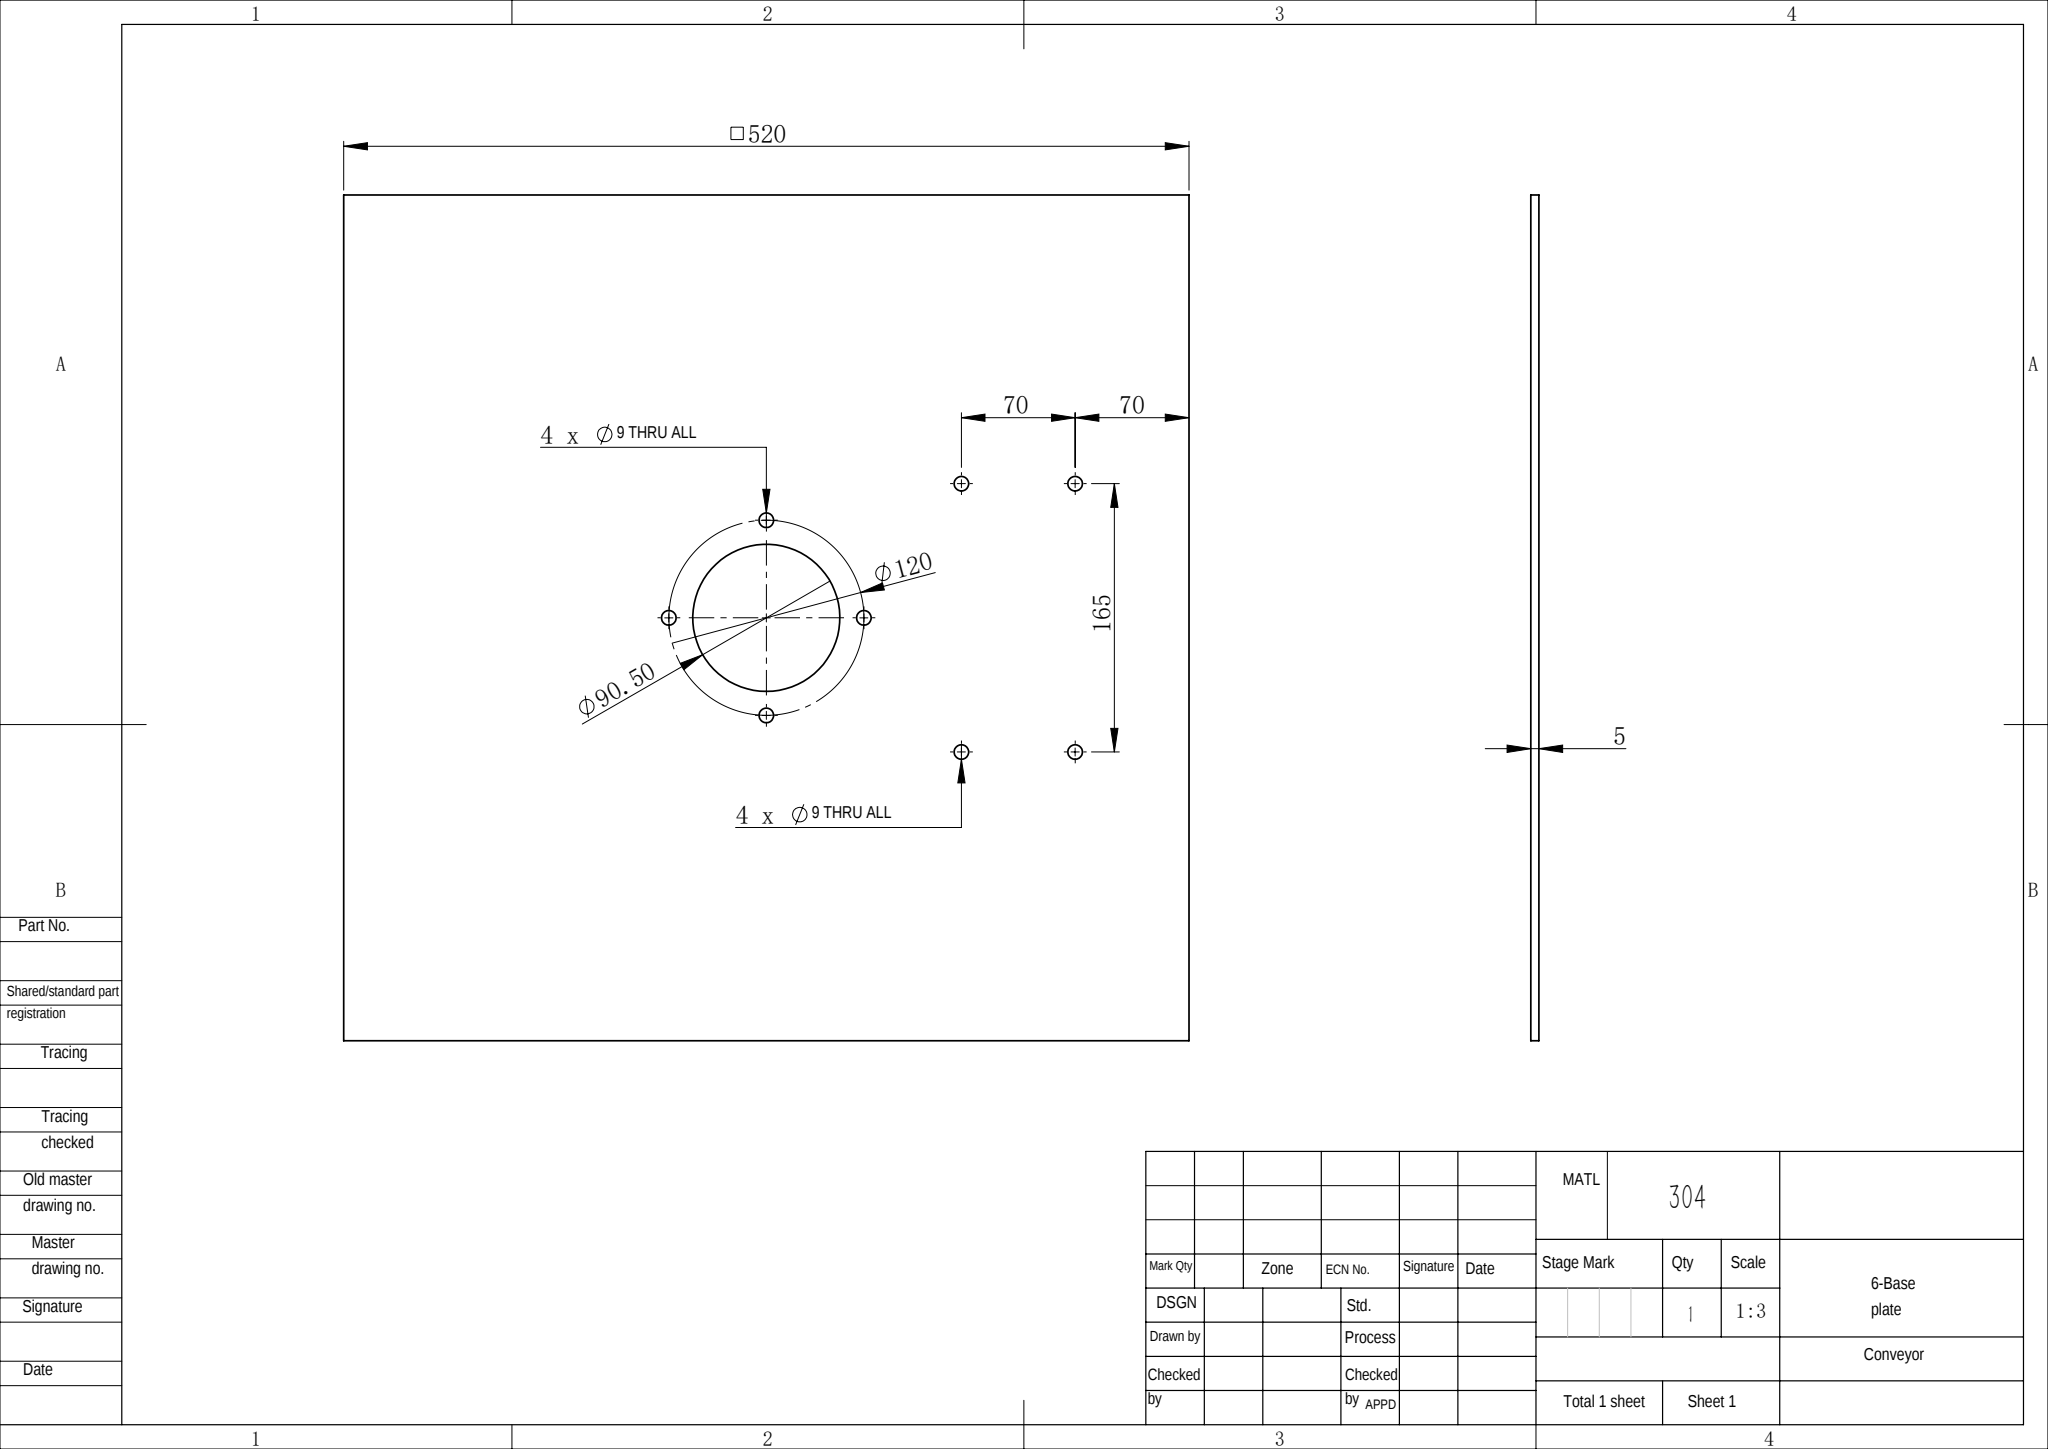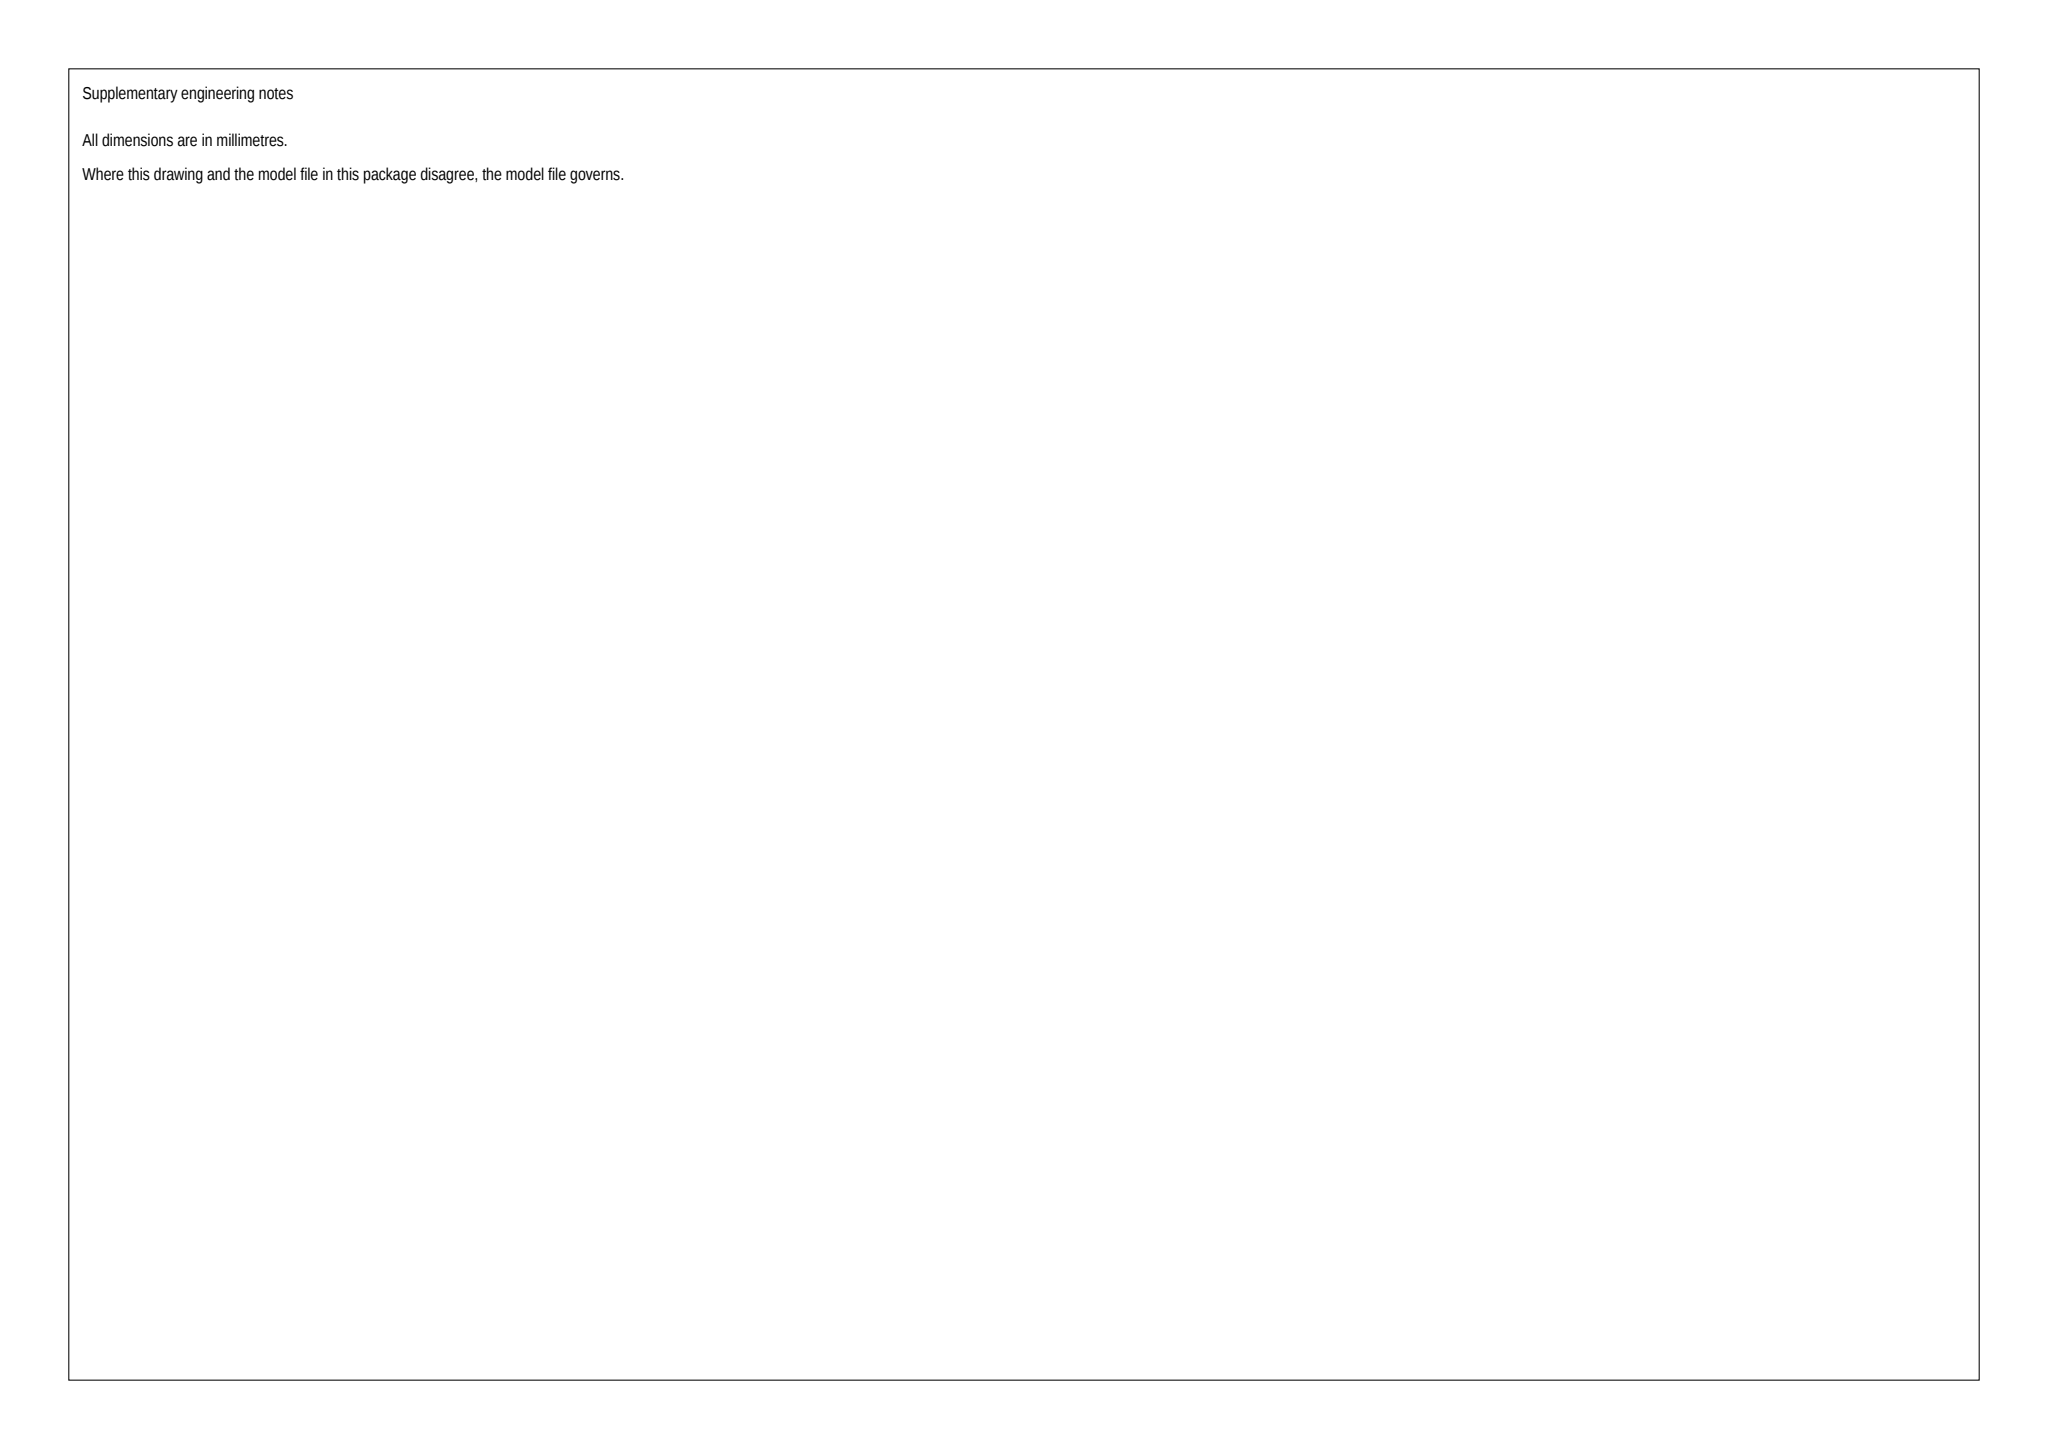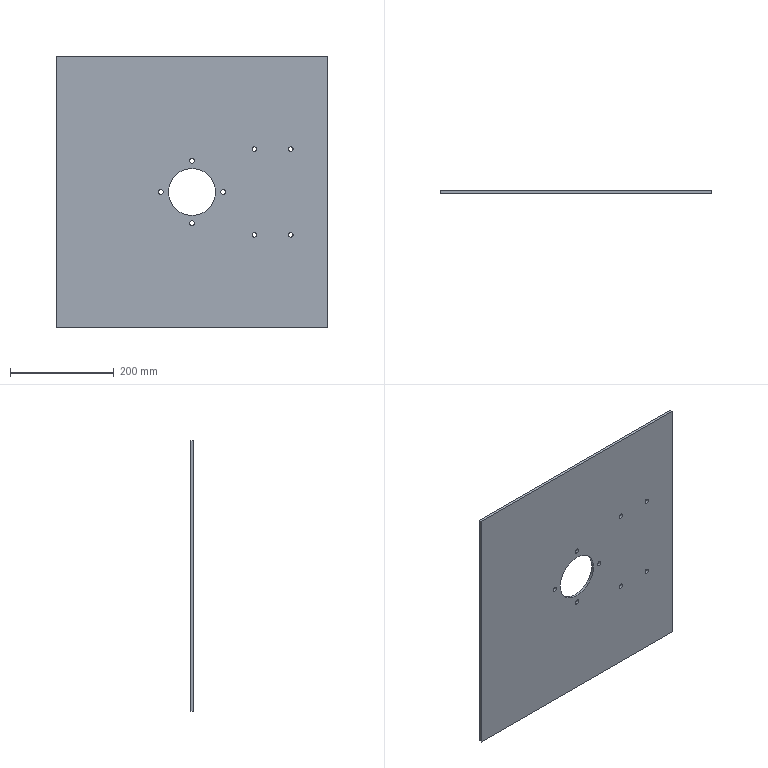Part | SolidWorks | mm | material 304 | 1 solid | 24 faces | box 520 x 5 x 520 mm | volume 1317292 mm3 | cylinder 18 | plane 6 | commonest cylinder face diameters 9 x16 90.5 x2
STEP:
#1=CARTESIAN_POINT('',(120.,-5.,-87.));
#2=VERTEX_POINT('',#1);
#3=CARTESIAN_POINT('',(120.,-5.,-78.));
#4=VERTEX_POINT('',#3);
#5=CARTESIAN_POINT('',(120.,-5.,-82.5));
#6=DIRECTION('',(0.,1.,0.));
#7=DIRECTION('',(0.,0.,1.));
#8=AXIS2_PLACEMENT_3D('',#5,#6,#7);
#9=CIRCLE('',#8,4.5);
#10=EDGE_CURVE('',#2,#4,#9,.T.);
#11=ORIENTED_EDGE('',*,*,#10,.F.);
#12=CARTESIAN_POINT('',(120.,-0.,-87.));
#13=VERTEX_POINT('',#12);
#14=CARTESIAN_POINT('',(120.,0.,-87.));
#15=DIRECTION('',(0.,1.,0.));
#16=VECTOR('',#15,1000.);
#17=LINE('',#14,#16);
#18=EDGE_CURVE('',#2,#13,#17,.T.);
#19=ORIENTED_EDGE('',*,*,#18,.T.);
#20=CARTESIAN_POINT('',(120.,-0.,-78.));
#21=VERTEX_POINT('',#20);
#22=CARTESIAN_POINT('',(120.,-0.,-82.5));
#23=DIRECTION('',(0.,1.,0.));
#24=DIRECTION('',(0.,0.,1.));
#25=AXIS2_PLACEMENT_3D('',#22,#23,#24);
#26=CIRCLE('',#25,4.5);
#27=EDGE_CURVE('',#13,#21,#26,.T.);
#28=ORIENTED_EDGE('',*,*,#27,.T.);
#29=CARTESIAN_POINT('',(120.,0.,-78.));
#30=DIRECTION('',(0.,1.,0.));
#31=VECTOR('',#30,1000.);
#32=LINE('',#29,#31);
#33=EDGE_CURVE('',#4,#21,#32,.T.);
#34=ORIENTED_EDGE('',*,*,#33,.F.);
#35=EDGE_LOOP('',(#11,#19,#28,#34));
#36=FACE_OUTER_BOUND('',#35,.T.);
#37=CARTESIAN_POINT('',(120.,0.,-82.5));
#38=DIRECTION('',(0.,1.,0.));
#39=DIRECTION('',(0.,0.,1.));
#40=AXIS2_PLACEMENT_3D('',#37,#38,#39);
#41=CYLINDRICAL_SURFACE('',#40,4.5);
#42=ADVANCED_FACE('',(#36),#41,.F.);
#43=CARTESIAN_POINT('',(190.,-5.,78.));
#44=VERTEX_POINT('',#43);
#45=CARTESIAN_POINT('',(190.,-5.,87.));
#46=VERTEX_POINT('',#45);
#47=CARTESIAN_POINT('',(190.,-5.,82.5));
#48=DIRECTION('',(0.,1.,0.));
#49=DIRECTION('',(0.,0.,1.));
#50=AXIS2_PLACEMENT_3D('',#47,#48,#49);
#51=CIRCLE('',#50,4.5);
#52=EDGE_CURVE('',#44,#46,#51,.T.);
#53=ORIENTED_EDGE('',*,*,#52,.F.);
#54=CARTESIAN_POINT('',(190.,-0.,78.));
#55=VERTEX_POINT('',#54);
#56=CARTESIAN_POINT('',(190.,0.,78.));
#57=DIRECTION('',(0.,1.,0.));
#58=VECTOR('',#57,1000.);
#59=LINE('',#56,#58);
#60=EDGE_CURVE('',#44,#55,#59,.T.);
#61=ORIENTED_EDGE('',*,*,#60,.T.);
#62=CARTESIAN_POINT('',(190.,-0.,87.));
#63=VERTEX_POINT('',#62);
#64=CARTESIAN_POINT('',(190.,-0.,82.5));
#65=DIRECTION('',(0.,1.,0.));
#66=DIRECTION('',(0.,0.,1.));
#67=AXIS2_PLACEMENT_3D('',#64,#65,#66);
#68=CIRCLE('',#67,4.5);
#69=EDGE_CURVE('',#55,#63,#68,.T.);
#70=ORIENTED_EDGE('',*,*,#69,.T.);
#71=CARTESIAN_POINT('',(190.,0.,87.));
#72=DIRECTION('',(0.,1.,0.));
#73=VECTOR('',#72,1000.);
#74=LINE('',#71,#73);
#75=EDGE_CURVE('',#46,#63,#74,.T.);
#76=ORIENTED_EDGE('',*,*,#75,.F.);
#77=EDGE_LOOP('',(#53,#61,#70,#76));
#78=FACE_OUTER_BOUND('',#77,.T.);
#79=CARTESIAN_POINT('',(190.,0.,82.5));
#80=DIRECTION('',(0.,1.,0.));
#81=DIRECTION('',(0.,0.,1.));
#82=AXIS2_PLACEMENT_3D('',#79,#80,#81);
#83=CYLINDRICAL_SURFACE('',#82,4.5);
#84=ADVANCED_FACE('',(#78),#83,.F.);
#85=CARTESIAN_POINT('',(190.,-5.,-87.));
#86=VERTEX_POINT('',#85);
#87=CARTESIAN_POINT('',(190.,-5.,-78.));
#88=VERTEX_POINT('',#87);
#89=CARTESIAN_POINT('',(190.,-5.,-82.5));
#90=DIRECTION('',(0.,1.,0.));
#91=DIRECTION('',(0.,0.,1.));
#92=AXIS2_PLACEMENT_3D('',#89,#90,#91);
#93=CIRCLE('',#92,4.5);
#94=EDGE_CURVE('',#86,#88,#93,.T.);
#95=ORIENTED_EDGE('',*,*,#94,.F.);
#96=CARTESIAN_POINT('',(190.,-0.,-87.));
#97=VERTEX_POINT('',#96);
#98=CARTESIAN_POINT('',(190.,0.,-87.));
#99=DIRECTION('',(0.,1.,0.));
#100=VECTOR('',#99,1000.);
#101=LINE('',#98,#100);
#102=EDGE_CURVE('',#86,#97,#101,.T.);
#103=ORIENTED_EDGE('',*,*,#102,.T.);
#104=CARTESIAN_POINT('',(190.,-0.,-78.));
#105=VERTEX_POINT('',#104);
#106=CARTESIAN_POINT('',(190.,-0.,-82.5));
#107=DIRECTION('',(0.,1.,0.));
#108=DIRECTION('',(0.,0.,1.));
#109=AXIS2_PLACEMENT_3D('',#106,#107,#108);
#110=CIRCLE('',#109,4.5);
#111=EDGE_CURVE('',#97,#105,#110,.T.);
#112=ORIENTED_EDGE('',*,*,#111,.T.);
#113=CARTESIAN_POINT('',(190.,0.,-78.));
#114=DIRECTION('',(0.,1.,0.));
#115=VECTOR('',#114,1000.);
#116=LINE('',#113,#115);
#117=EDGE_CURVE('',#88,#105,#116,.T.);
#118=ORIENTED_EDGE('',*,*,#117,.F.);
#119=EDGE_LOOP('',(#95,#103,#112,#118));
#120=FACE_OUTER_BOUND('',#119,.T.);
#121=CARTESIAN_POINT('',(190.,0.,-82.5));
#122=DIRECTION('',(0.,1.,0.));
#123=DIRECTION('',(0.,0.,1.));
#124=AXIS2_PLACEMENT_3D('',#121,#122,#123);
#125=CYLINDRICAL_SURFACE('',#124,4.5);
#126=ADVANCED_FACE('',(#120),#125,.F.);
#127=CARTESIAN_POINT('',(120.,-5.,78.));
#128=VERTEX_POINT('',#127);
#129=CARTESIAN_POINT('',(120.,-5.,87.));
#130=VERTEX_POINT('',#129);
#131=CARTESIAN_POINT('',(120.,-5.,82.5));
#132=DIRECTION('',(0.,1.,0.));
#133=DIRECTION('',(0.,0.,1.));
#134=AXIS2_PLACEMENT_3D('',#131,#132,#133);
#135=CIRCLE('',#134,4.5);
#136=EDGE_CURVE('',#128,#130,#135,.T.);
#137=ORIENTED_EDGE('',*,*,#136,.F.);
#138=CARTESIAN_POINT('',(120.,-0.,78.));
#139=VERTEX_POINT('',#138);
#140=CARTESIAN_POINT('',(120.,0.,78.));
#141=DIRECTION('',(0.,1.,0.));
#142=VECTOR('',#141,1000.);
#143=LINE('',#140,#142);
#144=EDGE_CURVE('',#128,#139,#143,.T.);
#145=ORIENTED_EDGE('',*,*,#144,.T.);
#146=CARTESIAN_POINT('',(120.,-0.,87.));
#147=VERTEX_POINT('',#146);
#148=CARTESIAN_POINT('',(120.,-0.,82.5));
#149=DIRECTION('',(0.,1.,0.));
#150=DIRECTION('',(0.,0.,1.));
#151=AXIS2_PLACEMENT_3D('',#148,#149,#150);
#152=CIRCLE('',#151,4.5);
#153=EDGE_CURVE('',#139,#147,#152,.T.);
#154=ORIENTED_EDGE('',*,*,#153,.T.);
#155=CARTESIAN_POINT('',(120.,0.,87.));
#156=DIRECTION('',(0.,1.,0.));
#157=VECTOR('',#156,1000.);
#158=LINE('',#155,#157);
#159=EDGE_CURVE('',#130,#147,#158,.T.);
#160=ORIENTED_EDGE('',*,*,#159,.F.);
#161=EDGE_LOOP('',(#137,#145,#154,#160));
#162=FACE_OUTER_BOUND('',#161,.T.);
#163=CARTESIAN_POINT('',(120.,0.,82.5));
#164=DIRECTION('',(0.,1.,0.));
#165=DIRECTION('',(0.,0.,1.));
#166=AXIS2_PLACEMENT_3D('',#163,#164,#165);
#167=CYLINDRICAL_SURFACE('',#166,4.5);
#168=ADVANCED_FACE('',(#162),#167,.F.);
#169=CARTESIAN_POINT('',(0.,-5.,-45.25));
#170=VERTEX_POINT('',#169);
#171=CARTESIAN_POINT('',(0.,-5.,45.25));
#172=VERTEX_POINT('',#171);
#173=CARTESIAN_POINT('',(0.,-5.,0.));
#174=DIRECTION('',(0.,1.,0.));
#175=DIRECTION('',(0.,0.,1.));
#176=AXIS2_PLACEMENT_3D('',#173,#174,#175);
#177=CIRCLE('',#176,45.25);
#178=EDGE_CURVE('',#170,#172,#177,.T.);
#179=ORIENTED_EDGE('',*,*,#178,.F.);
#180=CARTESIAN_POINT('',(0.,0.,-45.25));
#181=VERTEX_POINT('',#180);
#182=CARTESIAN_POINT('',(0.,-10.,-45.25));
#183=DIRECTION('',(0.,1.,0.));
#184=VECTOR('',#183,1000.);
#185=LINE('',#182,#184);
#186=EDGE_CURVE('',#170,#181,#185,.T.);
#187=ORIENTED_EDGE('',*,*,#186,.T.);
#188=CARTESIAN_POINT('',(0.,0.,45.25));
#189=VERTEX_POINT('',#188);
#190=CARTESIAN_POINT('',(0.,0.,0.));
#191=DIRECTION('',(0.,1.,0.));
#192=DIRECTION('',(0.,0.,1.));
#193=AXIS2_PLACEMENT_3D('',#190,#191,#192);
#194=CIRCLE('',#193,45.25);
#195=EDGE_CURVE('',#181,#189,#194,.T.);
#196=ORIENTED_EDGE('',*,*,#195,.T.);
#197=CARTESIAN_POINT('',(0.,-10.,45.25));
#198=DIRECTION('',(0.,1.,0.));
#199=VECTOR('',#198,1000.);
#200=LINE('',#197,#199);
#201=EDGE_CURVE('',#172,#189,#200,.T.);
#202=ORIENTED_EDGE('',*,*,#201,.F.);
#203=EDGE_LOOP('',(#179,#187,#196,#202));
#204=FACE_OUTER_BOUND('',#203,.T.);
#205=CARTESIAN_POINT('',(0.,-10.,0.));
#206=DIRECTION('',(0.,1.,0.));
#207=DIRECTION('',(0.,0.,1.));
#208=AXIS2_PLACEMENT_3D('',#205,#206,#207);
#209=CYLINDRICAL_SURFACE('',#208,45.25);
#210=ADVANCED_FACE('',(#204),#209,.F.);
#211=CARTESIAN_POINT('',(0.,-5.,-64.5));
#212=VERTEX_POINT('',#211);
#213=CARTESIAN_POINT('',(0.,-5.,-55.5));
#214=VERTEX_POINT('',#213);
#215=CARTESIAN_POINT('',(0.,-5.,-60.));
#216=DIRECTION('',(0.,1.,0.));
#217=DIRECTION('',(0.,0.,1.));
#218=AXIS2_PLACEMENT_3D('',#215,#216,#217);
#219=CIRCLE('',#218,4.5);
#220=EDGE_CURVE('',#212,#214,#219,.T.);
#221=ORIENTED_EDGE('',*,*,#220,.F.);
#222=CARTESIAN_POINT('',(0.,0.,-64.5));
#223=VERTEX_POINT('',#222);
#224=CARTESIAN_POINT('',(0.,0.,-64.5));
#225=DIRECTION('',(0.,1.,0.));
#226=VECTOR('',#225,1000.);
#227=LINE('',#224,#226);
#228=EDGE_CURVE('',#212,#223,#227,.T.);
#229=ORIENTED_EDGE('',*,*,#228,.T.);
#230=CARTESIAN_POINT('',(0.,0.,-55.5));
#231=VERTEX_POINT('',#230);
#232=CARTESIAN_POINT('',(0.,0.,-60.));
#233=DIRECTION('',(0.,1.,0.));
#234=DIRECTION('',(0.,0.,1.));
#235=AXIS2_PLACEMENT_3D('',#232,#233,#234);
#236=CIRCLE('',#235,4.5);
#237=EDGE_CURVE('',#223,#231,#236,.T.);
#238=ORIENTED_EDGE('',*,*,#237,.T.);
#239=CARTESIAN_POINT('',(0.,0.,-55.5));
#240=DIRECTION('',(0.,1.,0.));
#241=VECTOR('',#240,1000.);
#242=LINE('',#239,#241);
#243=EDGE_CURVE('',#214,#231,#242,.T.);
#244=ORIENTED_EDGE('',*,*,#243,.F.);
#245=EDGE_LOOP('',(#221,#229,#238,#244));
#246=FACE_OUTER_BOUND('',#245,.T.);
#247=CARTESIAN_POINT('',(0.,0.,-60.));
#248=DIRECTION('',(0.,1.,0.));
#249=DIRECTION('',(0.,0.,1.));
#250=AXIS2_PLACEMENT_3D('',#247,#248,#249);
#251=CYLINDRICAL_SURFACE('',#250,4.5);
#252=ADVANCED_FACE('',(#246),#251,.F.);
#253=CARTESIAN_POINT('',(-60.,-5.,-4.5));
#254=VERTEX_POINT('',#253);
#255=CARTESIAN_POINT('',(-60.,-5.,4.5));
#256=VERTEX_POINT('',#255);
#257=CARTESIAN_POINT('',(-60.,-5.,0.));
#258=DIRECTION('',(0.,1.,0.));
#259=DIRECTION('',(0.,0.,1.));
#260=AXIS2_PLACEMENT_3D('',#257,#258,#259);
#261=CIRCLE('',#260,4.5);
#262=EDGE_CURVE('',#254,#256,#261,.T.);
#263=ORIENTED_EDGE('',*,*,#262,.F.);
#264=CARTESIAN_POINT('',(-60.,0.,-4.5));
#265=VERTEX_POINT('',#264);
#266=CARTESIAN_POINT('',(-60.,0.,-4.5));
#267=DIRECTION('',(0.,1.,0.));
#268=VECTOR('',#267,1000.);
#269=LINE('',#266,#268);
#270=EDGE_CURVE('',#254,#265,#269,.T.);
#271=ORIENTED_EDGE('',*,*,#270,.T.);
#272=CARTESIAN_POINT('',(-60.,0.,4.5));
#273=VERTEX_POINT('',#272);
#274=CARTESIAN_POINT('',(-60.,0.,0.));
#275=DIRECTION('',(0.,1.,0.));
#276=DIRECTION('',(0.,0.,1.));
#277=AXIS2_PLACEMENT_3D('',#274,#275,#276);
#278=CIRCLE('',#277,4.5);
#279=EDGE_CURVE('',#265,#273,#278,.T.);
#280=ORIENTED_EDGE('',*,*,#279,.T.);
#281=CARTESIAN_POINT('',(-60.,0.,4.5));
#282=DIRECTION('',(0.,1.,0.));
#283=VECTOR('',#282,1000.);
#284=LINE('',#281,#283);
#285=EDGE_CURVE('',#256,#273,#284,.T.);
#286=ORIENTED_EDGE('',*,*,#285,.F.);
#287=EDGE_LOOP('',(#263,#271,#280,#286));
#288=FACE_OUTER_BOUND('',#287,.T.);
#289=CARTESIAN_POINT('',(-60.,0.,0.));
#290=DIRECTION('',(0.,1.,0.));
#291=DIRECTION('',(0.,0.,1.));
#292=AXIS2_PLACEMENT_3D('',#289,#290,#291);
#293=CYLINDRICAL_SURFACE('',#292,4.5);
#294=ADVANCED_FACE('',(#288),#293,.F.);
#295=CARTESIAN_POINT('',(0.,-5.,55.5));
#296=VERTEX_POINT('',#295);
#297=CARTESIAN_POINT('',(0.,-5.,64.5));
#298=VERTEX_POINT('',#297);
#299=CARTESIAN_POINT('',(0.,-5.,60.));
#300=DIRECTION('',(0.,1.,0.));
#301=DIRECTION('',(0.,0.,1.));
#302=AXIS2_PLACEMENT_3D('',#299,#300,#301);
#303=CIRCLE('',#302,4.5);
#304=EDGE_CURVE('',#296,#298,#303,.T.);
#305=ORIENTED_EDGE('',*,*,#304,.F.);
#306=CARTESIAN_POINT('',(0.,0.,55.5));
#307=VERTEX_POINT('',#306);
#308=CARTESIAN_POINT('',(0.,0.,55.5));
#309=DIRECTION('',(0.,1.,0.));
#310=VECTOR('',#309,1000.);
#311=LINE('',#308,#310);
#312=EDGE_CURVE('',#296,#307,#311,.T.);
#313=ORIENTED_EDGE('',*,*,#312,.T.);
#314=CARTESIAN_POINT('',(0.,0.,64.5));
#315=VERTEX_POINT('',#314);
#316=CARTESIAN_POINT('',(0.,0.,60.));
#317=DIRECTION('',(0.,1.,0.));
#318=DIRECTION('',(0.,0.,1.));
#319=AXIS2_PLACEMENT_3D('',#316,#317,#318);
#320=CIRCLE('',#319,4.5);
#321=EDGE_CURVE('',#307,#315,#320,.T.);
#322=ORIENTED_EDGE('',*,*,#321,.T.);
#323=CARTESIAN_POINT('',(0.,0.,64.5));
#324=DIRECTION('',(0.,1.,0.));
#325=VECTOR('',#324,1000.);
#326=LINE('',#323,#325);
#327=EDGE_CURVE('',#298,#315,#326,.T.);
#328=ORIENTED_EDGE('',*,*,#327,.F.);
#329=EDGE_LOOP('',(#305,#313,#322,#328));
#330=FACE_OUTER_BOUND('',#329,.T.);
#331=CARTESIAN_POINT('',(0.,0.,60.));
#332=DIRECTION('',(0.,1.,0.));
#333=DIRECTION('',(0.,0.,1.));
#334=AXIS2_PLACEMENT_3D('',#331,#332,#333);
#335=CYLINDRICAL_SURFACE('',#334,4.5);
#336=ADVANCED_FACE('',(#330),#335,.F.);
#337=CARTESIAN_POINT('',(60.,-5.,-4.5));
#338=VERTEX_POINT('',#337);
#339=CARTESIAN_POINT('',(60.,-5.,4.5));
#340=VERTEX_POINT('',#339);
#341=CARTESIAN_POINT('',(60.,-5.,0.));
#342=DIRECTION('',(0.,1.,0.));
#343=DIRECTION('',(0.,0.,1.));
#344=AXIS2_PLACEMENT_3D('',#341,#342,#343);
#345=CIRCLE('',#344,4.5);
#346=EDGE_CURVE('',#338,#340,#345,.T.);
#347=ORIENTED_EDGE('',*,*,#346,.F.);
#348=CARTESIAN_POINT('',(60.,0.,-4.5));
#349=VERTEX_POINT('',#348);
#350=CARTESIAN_POINT('',(60.,0.,-4.5));
#351=DIRECTION('',(0.,1.,0.));
#352=VECTOR('',#351,1000.);
#353=LINE('',#350,#352);
#354=EDGE_CURVE('',#338,#349,#353,.T.);
#355=ORIENTED_EDGE('',*,*,#354,.T.);
#356=CARTESIAN_POINT('',(60.,0.,4.5));
#357=VERTEX_POINT('',#356);
#358=CARTESIAN_POINT('',(60.,0.,0.));
#359=DIRECTION('',(0.,1.,0.));
#360=DIRECTION('',(0.,0.,1.));
#361=AXIS2_PLACEMENT_3D('',#358,#359,#360);
#362=CIRCLE('',#361,4.5);
#363=EDGE_CURVE('',#349,#357,#362,.T.);
#364=ORIENTED_EDGE('',*,*,#363,.T.);
#365=CARTESIAN_POINT('',(60.,0.,4.5));
#366=DIRECTION('',(0.,1.,0.));
#367=VECTOR('',#366,1000.);
#368=LINE('',#365,#367);
#369=EDGE_CURVE('',#340,#357,#368,.T.);
#370=ORIENTED_EDGE('',*,*,#369,.F.);
#371=EDGE_LOOP('',(#347,#355,#364,#370));
#372=FACE_OUTER_BOUND('',#371,.T.);
#373=CARTESIAN_POINT('',(60.,0.,0.));
#374=DIRECTION('',(0.,1.,0.));
#375=DIRECTION('',(0.,0.,1.));
#376=AXIS2_PLACEMENT_3D('',#373,#374,#375);
#377=CYLINDRICAL_SURFACE('',#376,4.5);
#378=ADVANCED_FACE('',(#372),#377,.F.);
#379=CARTESIAN_POINT('',(-260.,0.,-260.));
#380=VERTEX_POINT('',#379);
#381=CARTESIAN_POINT('',(-260.,0.,260.));
#382=VERTEX_POINT('',#381);
#383=CARTESIAN_POINT('',(-260.,0.,260.));
#384=DIRECTION('',(0.,0.,1.));
#385=VECTOR('',#384,1000.);
#386=LINE('',#383,#385);
#387=EDGE_CURVE('',#380,#382,#386,.T.);
#388=ORIENTED_EDGE('',*,*,#387,.F.);
#389=CARTESIAN_POINT('',(-260.,-5.,-260.));
#390=VERTEX_POINT('',#389);
#391=CARTESIAN_POINT('',(-260.,-5.,-260.));
#392=DIRECTION('',(0.,1.,0.));
#393=VECTOR('',#392,1000.);
#394=LINE('',#391,#393);
#395=EDGE_CURVE('',#390,#380,#394,.T.);
#396=ORIENTED_EDGE('',*,*,#395,.F.);
#397=CARTESIAN_POINT('',(-260.,-5.,260.));
#398=VERTEX_POINT('',#397);
#399=CARTESIAN_POINT('',(-260.,-5.,260.));
#400=DIRECTION('',(0.,0.,1.));
#401=VECTOR('',#400,1000.);
#402=LINE('',#399,#401);
#403=EDGE_CURVE('',#390,#398,#402,.T.);
#404=ORIENTED_EDGE('',*,*,#403,.T.);
#405=CARTESIAN_POINT('',(-260.,-5.,260.));
#406=DIRECTION('',(0.,1.,0.));
#407=VECTOR('',#406,1000.);
#408=LINE('',#405,#407);
#409=EDGE_CURVE('',#398,#382,#408,.T.);
#410=ORIENTED_EDGE('',*,*,#409,.T.);
#411=EDGE_LOOP('',(#388,#396,#404,#410));
#412=FACE_OUTER_BOUND('',#411,.T.);
#413=CARTESIAN_POINT('',(-260.,-5.,260.));
#414=DIRECTION('',(-1.,0.,0.));
#415=DIRECTION('',(0.,0.,1.));
#416=AXIS2_PLACEMENT_3D('',#413,#414,#415);
#417=PLANE('',#416);
#418=ADVANCED_FACE('',(#412),#417,.T.);
#419=CARTESIAN_POINT('',(260.,0.,-260.));
#420=VERTEX_POINT('',#419);
#421=CARTESIAN_POINT('',(260.,0.,-260.));
#422=DIRECTION('',(-1.,0.,0.));
#423=VECTOR('',#422,1000.);
#424=LINE('',#421,#423);
#425=EDGE_CURVE('',#420,#380,#424,.T.);
#426=ORIENTED_EDGE('',*,*,#425,.F.);
#427=CARTESIAN_POINT('',(260.,-5.,-260.));
#428=VERTEX_POINT('',#427);
#429=CARTESIAN_POINT('',(260.,-5.,-260.));
#430=DIRECTION('',(0.,1.,0.));
#431=VECTOR('',#430,1000.);
#432=LINE('',#429,#431);
#433=EDGE_CURVE('',#428,#420,#432,.T.);
#434=ORIENTED_EDGE('',*,*,#433,.F.);
#435=CARTESIAN_POINT('',(260.,-5.,-260.));
#436=DIRECTION('',(-1.,0.,0.));
#437=VECTOR('',#436,1000.);
#438=LINE('',#435,#437);
#439=EDGE_CURVE('',#428,#390,#438,.T.);
#440=ORIENTED_EDGE('',*,*,#439,.T.);
#441=ORIENTED_EDGE('',*,*,#395,.T.);
#442=EDGE_LOOP('',(#426,#434,#440,#441));
#443=FACE_OUTER_BOUND('',#442,.T.);
#444=CARTESIAN_POINT('',(260.,-5.,-260.));
#445=DIRECTION('',(-0.,0.,-1.));
#446=DIRECTION('',(-1.,0.,0.));
#447=AXIS2_PLACEMENT_3D('',#444,#445,#446);
#448=PLANE('',#447);
#449=ADVANCED_FACE('',(#443),#448,.T.);
#450=CARTESIAN_POINT('',(260.,0.,260.));
#451=VERTEX_POINT('',#450);
#452=CARTESIAN_POINT('',(260.,0.,260.));
#453=DIRECTION('',(0.,0.,-1.));
#454=VECTOR('',#453,1000.);
#455=LINE('',#452,#454);
#456=EDGE_CURVE('',#451,#420,#455,.T.);
#457=ORIENTED_EDGE('',*,*,#456,.F.);
#458=CARTESIAN_POINT('',(260.,-5.,260.));
#459=VERTEX_POINT('',#458);
#460=CARTESIAN_POINT('',(260.,-5.,260.));
#461=DIRECTION('',(0.,1.,0.));
#462=VECTOR('',#461,1000.);
#463=LINE('',#460,#462);
#464=EDGE_CURVE('',#459,#451,#463,.T.);
#465=ORIENTED_EDGE('',*,*,#464,.F.);
#466=CARTESIAN_POINT('',(260.,-5.,260.));
#467=DIRECTION('',(0.,0.,-1.));
#468=VECTOR('',#467,1000.);
#469=LINE('',#466,#468);
#470=EDGE_CURVE('',#459,#428,#469,.T.);
#471=ORIENTED_EDGE('',*,*,#470,.T.);
#472=ORIENTED_EDGE('',*,*,#433,.T.);
#473=EDGE_LOOP('',(#457,#465,#471,#472));
#474=FACE_OUTER_BOUND('',#473,.T.);
#475=CARTESIAN_POINT('',(260.,-5.,260.));
#476=DIRECTION('',(1.,0.,0.));
#477=DIRECTION('',(0.,0.,-1.));
#478=AXIS2_PLACEMENT_3D('',#475,#476,#477);
#479=PLANE('',#478);
#480=ADVANCED_FACE('',(#474),#479,.T.);
#481=CARTESIAN_POINT('',(260.,0.,260.));
#482=DIRECTION('',(1.,0.,-0.));
#483=VECTOR('',#482,1000.);
#484=LINE('',#481,#483);
#485=EDGE_CURVE('',#382,#451,#484,.T.);
#486=ORIENTED_EDGE('',*,*,#485,.F.);
#487=ORIENTED_EDGE('',*,*,#409,.F.);
#488=CARTESIAN_POINT('',(260.,-5.,260.));
#489=DIRECTION('',(1.,0.,-0.));
#490=VECTOR('',#489,1000.);
#491=LINE('',#488,#490);
#492=EDGE_CURVE('',#398,#459,#491,.T.);
#493=ORIENTED_EDGE('',*,*,#492,.T.);
#494=ORIENTED_EDGE('',*,*,#464,.T.);
#495=EDGE_LOOP('',(#486,#487,#493,#494));
#496=FACE_OUTER_BOUND('',#495,.T.);
#497=CARTESIAN_POINT('',(260.,-5.,260.));
#498=DIRECTION('',(0.,0.,1.));
#499=DIRECTION('',(1.,0.,-0.));
#500=AXIS2_PLACEMENT_3D('',#497,#498,#499);
#501=PLANE('',#500);
#502=ADVANCED_FACE('',(#496),#501,.T.);
#503=CARTESIAN_POINT('',(120.,-5.,-82.5));
#504=DIRECTION('',(0.,1.,0.));
#505=DIRECTION('',(0.,0.,1.));
#506=AXIS2_PLACEMENT_3D('',#503,#504,#505);
#507=CIRCLE('',#506,4.5);
#508=EDGE_CURVE('',#4,#2,#507,.T.);
#509=ORIENTED_EDGE('',*,*,#508,.T.);
#510=ORIENTED_EDGE('',*,*,#10,.T.);
#511=EDGE_LOOP('',(#509,#510));
#512=FACE_BOUND('',#511,.T.);
#513=CARTESIAN_POINT('',(190.,-5.,82.5));
#514=DIRECTION('',(0.,1.,0.));
#515=DIRECTION('',(0.,0.,1.));
#516=AXIS2_PLACEMENT_3D('',#513,#514,#515);
#517=CIRCLE('',#516,4.5);
#518=EDGE_CURVE('',#46,#44,#517,.T.);
#519=ORIENTED_EDGE('',*,*,#518,.T.);
#520=ORIENTED_EDGE('',*,*,#52,.T.);
#521=EDGE_LOOP('',(#519,#520));
#522=FACE_BOUND('',#521,.T.);
#523=CARTESIAN_POINT('',(190.,-5.,-82.5));
#524=DIRECTION('',(0.,1.,0.));
#525=DIRECTION('',(0.,0.,1.));
#526=AXIS2_PLACEMENT_3D('',#523,#524,#525);
#527=CIRCLE('',#526,4.5);
#528=EDGE_CURVE('',#88,#86,#527,.T.);
#529=ORIENTED_EDGE('',*,*,#528,.T.);
#530=ORIENTED_EDGE('',*,*,#94,.T.);
#531=EDGE_LOOP('',(#529,#530));
#532=FACE_BOUND('',#531,.T.);
#533=CARTESIAN_POINT('',(120.,-5.,82.5));
#534=DIRECTION('',(0.,1.,0.));
#535=DIRECTION('',(0.,0.,1.));
#536=AXIS2_PLACEMENT_3D('',#533,#534,#535);
#537=CIRCLE('',#536,4.5);
#538=EDGE_CURVE('',#130,#128,#537,.T.);
#539=ORIENTED_EDGE('',*,*,#538,.T.);
#540=ORIENTED_EDGE('',*,*,#136,.T.);
#541=EDGE_LOOP('',(#539,#540));
#542=FACE_BOUND('',#541,.T.);
#543=CARTESIAN_POINT('',(0.,-5.,0.));
#544=DIRECTION('',(0.,1.,0.));
#545=DIRECTION('',(0.,0.,1.));
#546=AXIS2_PLACEMENT_3D('',#543,#544,#545);
#547=CIRCLE('',#546,45.25);
#548=EDGE_CURVE('',#172,#170,#547,.T.);
#549=ORIENTED_EDGE('',*,*,#548,.T.);
#550=ORIENTED_EDGE('',*,*,#178,.T.);
#551=EDGE_LOOP('',(#549,#550));
#552=FACE_BOUND('',#551,.T.);
#553=CARTESIAN_POINT('',(0.,-5.,-60.));
#554=DIRECTION('',(0.,1.,0.));
#555=DIRECTION('',(0.,0.,1.));
#556=AXIS2_PLACEMENT_3D('',#553,#554,#555);
#557=CIRCLE('',#556,4.5);
#558=EDGE_CURVE('',#214,#212,#557,.T.);
#559=ORIENTED_EDGE('',*,*,#558,.T.);
#560=ORIENTED_EDGE('',*,*,#220,.T.);
#561=EDGE_LOOP('',(#559,#560));
#562=FACE_BOUND('',#561,.T.);
#563=CARTESIAN_POINT('',(-60.,-5.,0.));
#564=DIRECTION('',(0.,1.,0.));
#565=DIRECTION('',(0.,0.,1.));
#566=AXIS2_PLACEMENT_3D('',#563,#564,#565);
#567=CIRCLE('',#566,4.5);
#568=EDGE_CURVE('',#256,#254,#567,.T.);
#569=ORIENTED_EDGE('',*,*,#568,.T.);
#570=ORIENTED_EDGE('',*,*,#262,.T.);
#571=EDGE_LOOP('',(#569,#570));
#572=FACE_BOUND('',#571,.T.);
#573=CARTESIAN_POINT('',(0.,-5.,60.));
#574=DIRECTION('',(0.,1.,0.));
#575=DIRECTION('',(0.,0.,1.));
#576=AXIS2_PLACEMENT_3D('',#573,#574,#575);
#577=CIRCLE('',#576,4.5);
#578=EDGE_CURVE('',#298,#296,#577,.T.);
#579=ORIENTED_EDGE('',*,*,#578,.T.);
#580=ORIENTED_EDGE('',*,*,#304,.T.);
#581=EDGE_LOOP('',(#579,#580));
#582=FACE_BOUND('',#581,.T.);
#583=CARTESIAN_POINT('',(60.,-5.,0.));
#584=DIRECTION('',(0.,1.,0.));
#585=DIRECTION('',(0.,0.,1.));
#586=AXIS2_PLACEMENT_3D('',#583,#584,#585);
#587=CIRCLE('',#586,4.5);
#588=EDGE_CURVE('',#340,#338,#587,.T.);
#589=ORIENTED_EDGE('',*,*,#588,.T.);
#590=ORIENTED_EDGE('',*,*,#346,.T.);
#591=EDGE_LOOP('',(#589,#590));
#592=FACE_BOUND('',#591,.T.);
#593=ORIENTED_EDGE('',*,*,#403,.F.);
#594=ORIENTED_EDGE('',*,*,#439,.F.);
#595=ORIENTED_EDGE('',*,*,#470,.F.);
#596=ORIENTED_EDGE('',*,*,#492,.F.);
#597=EDGE_LOOP('',(#593,#594,#595,#596));
#598=FACE_OUTER_BOUND('',#597,.T.);
#599=CARTESIAN_POINT('',(0.,-5.,0.));
#600=DIRECTION('',(0.,1.,0.));
#601=DIRECTION('',(0.,0.,1.));
#602=AXIS2_PLACEMENT_3D('',#599,#600,#601);
#603=PLANE('',#602);
#604=ADVANCED_FACE('',(#512,#522,#532,#542,#552,#562,#572,#582,#592,#598),#603,.F.);
#605=CARTESIAN_POINT('',(120.,-0.,-82.5));
#606=DIRECTION('',(0.,1.,0.));
#607=DIRECTION('',(0.,0.,1.));
#608=AXIS2_PLACEMENT_3D('',#605,#606,#607);
#609=CIRCLE('',#608,4.5);
#610=EDGE_CURVE('',#21,#13,#609,.T.);
#611=ORIENTED_EDGE('',*,*,#610,.F.);
#612=ORIENTED_EDGE('',*,*,#27,.F.);
#613=EDGE_LOOP('',(#611,#612));
#614=FACE_BOUND('',#613,.T.);
#615=CARTESIAN_POINT('',(190.,-0.,82.5));
#616=DIRECTION('',(0.,1.,0.));
#617=DIRECTION('',(0.,0.,1.));
#618=AXIS2_PLACEMENT_3D('',#615,#616,#617);
#619=CIRCLE('',#618,4.5);
#620=EDGE_CURVE('',#63,#55,#619,.T.);
#621=ORIENTED_EDGE('',*,*,#620,.F.);
#622=ORIENTED_EDGE('',*,*,#69,.F.);
#623=EDGE_LOOP('',(#621,#622));
#624=FACE_BOUND('',#623,.T.);
#625=CARTESIAN_POINT('',(190.,-0.,-82.5));
#626=DIRECTION('',(0.,1.,0.));
#627=DIRECTION('',(0.,0.,1.));
#628=AXIS2_PLACEMENT_3D('',#625,#626,#627);
#629=CIRCLE('',#628,4.5);
#630=EDGE_CURVE('',#105,#97,#629,.T.);
#631=ORIENTED_EDGE('',*,*,#630,.F.);
#632=ORIENTED_EDGE('',*,*,#111,.F.);
#633=EDGE_LOOP('',(#631,#632));
#634=FACE_BOUND('',#633,.T.);
#635=CARTESIAN_POINT('',(120.,-0.,82.5));
#636=DIRECTION('',(0.,1.,0.));
#637=DIRECTION('',(0.,0.,1.));
#638=AXIS2_PLACEMENT_3D('',#635,#636,#637);
#639=CIRCLE('',#638,4.5);
#640=EDGE_CURVE('',#147,#139,#639,.T.);
#641=ORIENTED_EDGE('',*,*,#640,.F.);
#642=ORIENTED_EDGE('',*,*,#153,.F.);
#643=EDGE_LOOP('',(#641,#642));
#644=FACE_BOUND('',#643,.T.);
#645=CARTESIAN_POINT('',(0.,0.,0.));
#646=DIRECTION('',(0.,1.,0.));
#647=DIRECTION('',(0.,0.,1.));
#648=AXIS2_PLACEMENT_3D('',#645,#646,#647);
#649=CIRCLE('',#648,45.25);
#650=EDGE_CURVE('',#189,#181,#649,.T.);
#651=ORIENTED_EDGE('',*,*,#650,.F.);
#652=ORIENTED_EDGE('',*,*,#195,.F.);
#653=EDGE_LOOP('',(#651,#652));
#654=FACE_BOUND('',#653,.T.);
#655=CARTESIAN_POINT('',(0.,0.,-60.));
#656=DIRECTION('',(0.,1.,0.));
#657=DIRECTION('',(0.,0.,1.));
#658=AXIS2_PLACEMENT_3D('',#655,#656,#657);
#659=CIRCLE('',#658,4.5);
#660=EDGE_CURVE('',#231,#223,#659,.T.);
#661=ORIENTED_EDGE('',*,*,#660,.F.);
#662=ORIENTED_EDGE('',*,*,#237,.F.);
#663=EDGE_LOOP('',(#661,#662));
#664=FACE_BOUND('',#663,.T.);
#665=CARTESIAN_POINT('',(-60.,0.,0.));
#666=DIRECTION('',(0.,1.,0.));
#667=DIRECTION('',(0.,0.,1.));
#668=AXIS2_PLACEMENT_3D('',#665,#666,#667);
#669=CIRCLE('',#668,4.5);
#670=EDGE_CURVE('',#273,#265,#669,.T.);
#671=ORIENTED_EDGE('',*,*,#670,.F.);
#672=ORIENTED_EDGE('',*,*,#279,.F.);
#673=EDGE_LOOP('',(#671,#672));
#674=FACE_BOUND('',#673,.T.);
#675=CARTESIAN_POINT('',(0.,0.,60.));
#676=DIRECTION('',(0.,1.,0.));
#677=DIRECTION('',(0.,0.,1.));
#678=AXIS2_PLACEMENT_3D('',#675,#676,#677);
#679=CIRCLE('',#678,4.5);
#680=EDGE_CURVE('',#315,#307,#679,.T.);
#681=ORIENTED_EDGE('',*,*,#680,.F.);
#682=ORIENTED_EDGE('',*,*,#321,.F.);
#683=EDGE_LOOP('',(#681,#682));
#684=FACE_BOUND('',#683,.T.);
#685=CARTESIAN_POINT('',(60.,0.,0.));
#686=DIRECTION('',(0.,1.,0.));
#687=DIRECTION('',(0.,0.,1.));
#688=AXIS2_PLACEMENT_3D('',#685,#686,#687);
#689=CIRCLE('',#688,4.5);
#690=EDGE_CURVE('',#357,#349,#689,.T.);
#691=ORIENTED_EDGE('',*,*,#690,.F.);
#692=ORIENTED_EDGE('',*,*,#363,.F.);
#693=EDGE_LOOP('',(#691,#692));
#694=FACE_BOUND('',#693,.T.);
#695=ORIENTED_EDGE('',*,*,#387,.T.);
#696=ORIENTED_EDGE('',*,*,#485,.T.);
#697=ORIENTED_EDGE('',*,*,#456,.T.);
#698=ORIENTED_EDGE('',*,*,#425,.T.);
#699=EDGE_LOOP('',(#695,#696,#697,#698));
#700=FACE_OUTER_BOUND('',#699,.T.);
#701=CARTESIAN_POINT('',(0.,0.,0.));
#702=DIRECTION('',(0.,1.,0.));
#703=DIRECTION('',(0.,0.,1.));
#704=AXIS2_PLACEMENT_3D('',#701,#702,#703);
#705=PLANE('',#704);
#706=ADVANCED_FACE('',(#614,#624,#634,#644,#654,#664,#674,#684,#694,#700),#705,.T.);
#707=ORIENTED_EDGE('',*,*,#354,.F.);
#708=ORIENTED_EDGE('',*,*,#588,.F.);
#709=ORIENTED_EDGE('',*,*,#369,.T.);
#710=ORIENTED_EDGE('',*,*,#690,.T.);
#711=EDGE_LOOP('',(#707,#708,#709,#710));
#712=FACE_OUTER_BOUND('',#711,.T.);
#713=CARTESIAN_POINT('',(60.,0.,0.));
#714=DIRECTION('',(0.,1.,0.));
#715=DIRECTION('',(0.,0.,1.));
#716=AXIS2_PLACEMENT_3D('',#713,#714,#715);
#717=CYLINDRICAL_SURFACE('',#716,4.5);
#718=ADVANCED_FACE('',(#712),#717,.F.);
#719=ORIENTED_EDGE('',*,*,#312,.F.);
#720=ORIENTED_EDGE('',*,*,#578,.F.);
#721=ORIENTED_EDGE('',*,*,#327,.T.);
#722=ORIENTED_EDGE('',*,*,#680,.T.);
#723=EDGE_LOOP('',(#719,#720,#721,#722));
#724=FACE_OUTER_BOUND('',#723,.T.);
#725=CARTESIAN_POINT('',(0.,0.,60.));
#726=DIRECTION('',(0.,1.,0.));
#727=DIRECTION('',(0.,0.,1.));
#728=AXIS2_PLACEMENT_3D('',#725,#726,#727);
#729=CYLINDRICAL_SURFACE('',#728,4.5);
#730=ADVANCED_FACE('',(#724),#729,.F.);
#731=ORIENTED_EDGE('',*,*,#270,.F.);
#732=ORIENTED_EDGE('',*,*,#568,.F.);
#733=ORIENTED_EDGE('',*,*,#285,.T.);
#734=ORIENTED_EDGE('',*,*,#670,.T.);
#735=EDGE_LOOP('',(#731,#732,#733,#734));
#736=FACE_OUTER_BOUND('',#735,.T.);
#737=CARTESIAN_POINT('',(-60.,0.,0.));
#738=DIRECTION('',(0.,1.,0.));
#739=DIRECTION('',(0.,0.,1.));
#740=AXIS2_PLACEMENT_3D('',#737,#738,#739);
#741=CYLINDRICAL_SURFACE('',#740,4.5);
#742=ADVANCED_FACE('',(#736),#741,.F.);
#743=ORIENTED_EDGE('',*,*,#228,.F.);
#744=ORIENTED_EDGE('',*,*,#558,.F.);
#745=ORIENTED_EDGE('',*,*,#243,.T.);
#746=ORIENTED_EDGE('',*,*,#660,.T.);
#747=EDGE_LOOP('',(#743,#744,#745,#746));
#748=FACE_OUTER_BOUND('',#747,.T.);
#749=CARTESIAN_POINT('',(0.,0.,-60.));
#750=DIRECTION('',(0.,1.,0.));
#751=DIRECTION('',(0.,0.,1.));
#752=AXIS2_PLACEMENT_3D('',#749,#750,#751);
#753=CYLINDRICAL_SURFACE('',#752,4.5);
#754=ADVANCED_FACE('',(#748),#753,.F.);
#755=ORIENTED_EDGE('',*,*,#186,.F.);
#756=ORIENTED_EDGE('',*,*,#548,.F.);
#757=ORIENTED_EDGE('',*,*,#201,.T.);
#758=ORIENTED_EDGE('',*,*,#650,.T.);
#759=EDGE_LOOP('',(#755,#756,#757,#758));
#760=FACE_OUTER_BOUND('',#759,.T.);
#761=CARTESIAN_POINT('',(0.,-10.,0.));
#762=DIRECTION('',(0.,1.,0.));
#763=DIRECTION('',(0.,0.,1.));
#764=AXIS2_PLACEMENT_3D('',#761,#762,#763);
#765=CYLINDRICAL_SURFACE('',#764,45.25);
#766=ADVANCED_FACE('',(#760),#765,.F.);
#767=ORIENTED_EDGE('',*,*,#144,.F.);
#768=ORIENTED_EDGE('',*,*,#538,.F.);
#769=ORIENTED_EDGE('',*,*,#159,.T.);
#770=ORIENTED_EDGE('',*,*,#640,.T.);
#771=EDGE_LOOP('',(#767,#768,#769,#770));
#772=FACE_OUTER_BOUND('',#771,.T.);
#773=CARTESIAN_POINT('',(120.,0.,82.5));
#774=DIRECTION('',(0.,1.,0.));
#775=DIRECTION('',(0.,0.,1.));
#776=AXIS2_PLACEMENT_3D('',#773,#774,#775);
#777=CYLINDRICAL_SURFACE('',#776,4.5);
#778=ADVANCED_FACE('',(#772),#777,.F.);
#779=ORIENTED_EDGE('',*,*,#102,.F.);
#780=ORIENTED_EDGE('',*,*,#528,.F.);
#781=ORIENTED_EDGE('',*,*,#117,.T.);
#782=ORIENTED_EDGE('',*,*,#630,.T.);
#783=EDGE_LOOP('',(#779,#780,#781,#782));
#784=FACE_OUTER_BOUND('',#783,.T.);
#785=CARTESIAN_POINT('',(190.,0.,-82.5));
#786=DIRECTION('',(0.,1.,0.));
#787=DIRECTION('',(0.,0.,1.));
#788=AXIS2_PLACEMENT_3D('',#785,#786,#787);
#789=CYLINDRICAL_SURFACE('',#788,4.5);
#790=ADVANCED_FACE('',(#784),#789,.F.);
#791=ORIENTED_EDGE('',*,*,#60,.F.);
#792=ORIENTED_EDGE('',*,*,#518,.F.);
#793=ORIENTED_EDGE('',*,*,#75,.T.);
#794=ORIENTED_EDGE('',*,*,#620,.T.);
#795=EDGE_LOOP('',(#791,#792,#793,#794));
#796=FACE_OUTER_BOUND('',#795,.T.);
#797=CARTESIAN_POINT('',(190.,0.,82.5));
#798=DIRECTION('',(0.,1.,0.));
#799=DIRECTION('',(0.,0.,1.));
#800=AXIS2_PLACEMENT_3D('',#797,#798,#799);
#801=CYLINDRICAL_SURFACE('',#800,4.5);
#802=ADVANCED_FACE('',(#796),#801,.F.);
#803=ORIENTED_EDGE('',*,*,#18,.F.);
#804=ORIENTED_EDGE('',*,*,#508,.F.);
#805=ORIENTED_EDGE('',*,*,#33,.T.);
#806=ORIENTED_EDGE('',*,*,#610,.T.);
#807=EDGE_LOOP('',(#803,#804,#805,#806));
#808=FACE_OUTER_BOUND('',#807,.T.);
#809=CARTESIAN_POINT('',(120.,0.,-82.5));
#810=DIRECTION('',(0.,1.,0.));
#811=DIRECTION('',(0.,0.,1.));
#812=AXIS2_PLACEMENT_3D('',#809,#810,#811);
#813=CYLINDRICAL_SURFACE('',#812,4.5);
#814=ADVANCED_FACE('',(#808),#813,.F.);
#815=CLOSED_SHELL('',(#42,#84,#126,#168,#210,#252,#294,#336,#378,#418,#449,#480,#502,#604,#706,#718,#730,#742,#754,#766,#778,#790,#802,#814));
#816=MANIFOLD_SOLID_BREP('',#815);
#817=CARTESIAN_POINT('',(0.,0.,0.));
#818=DIRECTION('',(0.,0.,1.));
#819=DIRECTION('',(1.,0.,0.));
#820=AXIS2_PLACEMENT_3D('',#817,#818,#819);
#821=(LENGTH_UNIT()NAMED_UNIT(*)SI_UNIT(.MILLI.,.METRE.));
#822=UNCERTAINTY_MEASURE_WITH_UNIT(LENGTH_MEASURE(0.00001),#821,'','');
#823=(NAMED_UNIT(*)PLANE_ANGLE_UNIT()SI_UNIT($,.RADIAN.));
#824=(NAMED_UNIT(*)SI_UNIT($,.STERADIAN.)SOLID_ANGLE_UNIT());
#825=(GEOMETRIC_REPRESENTATION_CONTEXT(3)GLOBAL_UNCERTAINTY_ASSIGNED_CONTEXT((#822))GLOBAL_UNIT_ASSIGNED_CONTEXT((#821,#823,#824))REPRESENTATION_CONTEXT('',''));
#826=ADVANCED_BREP_SHAPE_REPRESENTATION('',(#816,#820),#825);